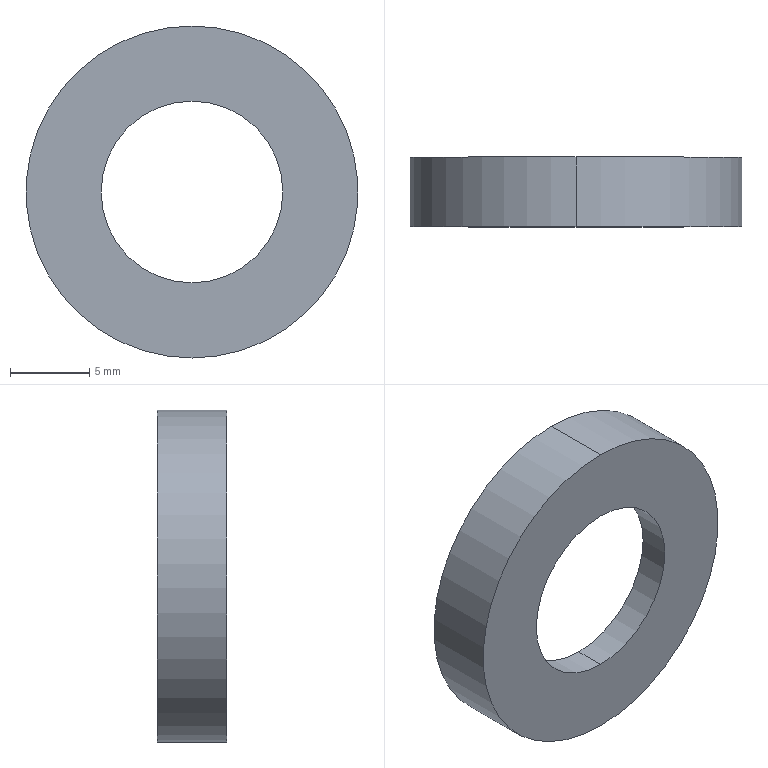Component | SolidWorks | SphericalWasherB21-1 | 1 solid | 8 faces | box 21 x 4.4 x 21 mm | volume 832 mm3 | cylinder 4 | cone 2 | plane 2 | commonest cylinder face diameters 21 x2 11.5 x2 | material Nickel
build123d program:
from build123d import *


with BuildPart() as part:
    # Sketch1 → Base-Revolve (revolve)
    with BuildSketch(Plane.XY, mode=Mode.PRIVATE) as base_revolve_sk:
        Polygon((5.75, 0), (10.5, 0), (10.5, 4.4), (10, 4.4), (5.75, 1.946), align=None)
    revolve(base_revolve_sk.sketch.rotate(Axis((0, 10.019, 0), (0, -1, 0)), 90), axis=Axis((0, 10.019, 0), (0, -1, 0)))


solid = part.part

# Placed as in the assembly
solid = solid.moved(Location((96, 228.606, 0), (0, 0, 0)))
STEP:
#1=COLOUR_RGB('',0.7922,0.8196,0.9333);
#2=FILL_AREA_STYLE_COLOUR('',#1);
#3=FILL_AREA_STYLE('',(#2));
#4=SURFACE_STYLE_FILL_AREA(#3);
#5=SURFACE_SIDE_STYLE('',(#4));
#6=SURFACE_STYLE_USAGE(.BOTH.,#5);
#7=PRESENTATION_STYLE_ASSIGNMENT((#6));
#8=CARTESIAN_POINT('',(3.78,9.077,-0.2264));
#9=VERTEX_POINT('',#8);
#10=CARTESIAN_POINT('',(3.78,9.077,0.2264));
#11=VERTEX_POINT('',#10);
#12=CARTESIAN_POINT('',(3.78,9.077,0.));
#13=DIRECTION('',(0.,1.,0.));
#14=DIRECTION('',(0.,0.,1.));
#15=AXIS2_PLACEMENT_3D('',#12,#13,#14);
#16=CIRCLE('',#15,0.2264);
#17=EDGE_CURVE('',#9,#11,#16,.T.);
#18=ORIENTED_EDGE('',*,*,#17,.F.);
#19=CARTESIAN_POINT('',(3.78,9.173,-0.3937));
#20=VERTEX_POINT('',#19);
#21=CARTESIAN_POINT('',(3.78,9.173,-0.3937));
#22=DIRECTION('',(0.,0.5,-0.866));
#23=VECTOR('',#22,39.37);
#24=LINE('',#21,#23);
#25=EDGE_CURVE('',#9,#20,#24,.T.);
#26=ORIENTED_EDGE('',*,*,#25,.T.);
#27=CARTESIAN_POINT('',(3.78,9.173,0.3937));
#28=VERTEX_POINT('',#27);
#29=CARTESIAN_POINT('',(3.78,9.173,0.));
#30=DIRECTION('',(0.,1.,0.));
#31=DIRECTION('',(0.,0.,1.));
#32=AXIS2_PLACEMENT_3D('',#29,#30,#31);
#33=CIRCLE('',#32,0.3937);
#34=EDGE_CURVE('',#20,#28,#33,.T.);
#35=ORIENTED_EDGE('',*,*,#34,.T.);
#36=CARTESIAN_POINT('',(3.78,9.173,0.3937));
#37=DIRECTION('',(0.,0.5,0.866));
#38=VECTOR('',#37,39.37);
#39=LINE('',#36,#38);
#40=EDGE_CURVE('',#11,#28,#39,.T.);
#41=ORIENTED_EDGE('',*,*,#40,.F.);
#42=EDGE_LOOP('',(#18,#26,#35,#41));
#43=FACE_OUTER_BOUND('',#42,.T.);
#44=CARTESIAN_POINT('',(3.78,9.173,0.));
#45=DIRECTION('',(0.,1.,0.));
#46=DIRECTION('',(0.,0.,1.));
#47=AXIS2_PLACEMENT_3D('',#44,#45,#46);
#48=CONICAL_SURFACE('',#47,0.3937,1.047);
#49=ADVANCED_FACE('',(#43),#48,.F.);
#50=CARTESIAN_POINT('',(3.78,9.,0.4134));
#51=VERTEX_POINT('',#50);
#52=CARTESIAN_POINT('',(3.78,9.,-0.4134));
#53=VERTEX_POINT('',#52);
#54=CARTESIAN_POINT('',(3.78,9.,0.));
#55=DIRECTION('',(0.,1.,0.));
#56=DIRECTION('',(0.,0.,1.));
#57=AXIS2_PLACEMENT_3D('',#54,#55,#56);
#58=CIRCLE('',#57,0.4134);
#59=EDGE_CURVE('',#51,#53,#58,.T.);
#60=ORIENTED_EDGE('',*,*,#59,.T.);
#61=CARTESIAN_POINT('',(3.78,9.173,-0.4134));
#62=VERTEX_POINT('',#61);
#63=CARTESIAN_POINT('',(3.78,9.395,-0.4134));
#64=DIRECTION('',(0.,1.,0.));
#65=VECTOR('',#64,39.37);
#66=LINE('',#63,#65);
#67=EDGE_CURVE('',#53,#62,#66,.T.);
#68=ORIENTED_EDGE('',*,*,#67,.T.);
#69=CARTESIAN_POINT('',(3.78,9.173,0.4134));
#70=VERTEX_POINT('',#69);
#71=CARTESIAN_POINT('',(3.78,9.173,0.));
#72=DIRECTION('',(0.,1.,0.));
#73=DIRECTION('',(0.,0.,1.));
#74=AXIS2_PLACEMENT_3D('',#71,#72,#73);
#75=CIRCLE('',#74,0.4134);
#76=EDGE_CURVE('',#70,#62,#75,.T.);
#77=ORIENTED_EDGE('',*,*,#76,.F.);
#78=CARTESIAN_POINT('',(3.78,9.395,0.4134));
#79=DIRECTION('',(0.,1.,0.));
#80=VECTOR('',#79,39.37);
#81=LINE('',#78,#80);
#82=EDGE_CURVE('',#51,#70,#81,.T.);
#83=ORIENTED_EDGE('',*,*,#82,.F.);
#84=EDGE_LOOP('',(#60,#68,#77,#83));
#85=FACE_OUTER_BOUND('',#84,.T.);
#86=CARTESIAN_POINT('',(3.78,9.395,0.));
#87=DIRECTION('',(0.,1.,0.));
#88=DIRECTION('',(0.,0.,1.));
#89=AXIS2_PLACEMENT_3D('',#86,#87,#88);
#90=CYLINDRICAL_SURFACE('',#89,0.4134);
#91=ADVANCED_FACE('',(#85),#90,.T.);
#92=CARTESIAN_POINT('',(3.78,9.,-0.2264));
#93=VERTEX_POINT('',#92);
#94=CARTESIAN_POINT('',(3.78,9.,0.2264));
#95=VERTEX_POINT('',#94);
#96=CARTESIAN_POINT('',(3.78,9.,0.));
#97=DIRECTION('',(0.,1.,0.));
#98=DIRECTION('',(0.,0.,1.));
#99=AXIS2_PLACEMENT_3D('',#96,#97,#98);
#100=CIRCLE('',#99,0.2264);
#101=EDGE_CURVE('',#93,#95,#100,.T.);
#102=ORIENTED_EDGE('',*,*,#101,.F.);
#103=CARTESIAN_POINT('',(3.78,9.395,-0.2264));
#104=DIRECTION('',(0.,1.,0.));
#105=VECTOR('',#104,39.37);
#106=LINE('',#103,#105);
#107=EDGE_CURVE('',#93,#9,#106,.T.);
#108=ORIENTED_EDGE('',*,*,#107,.T.);
#109=ORIENTED_EDGE('',*,*,#17,.T.);
#110=CARTESIAN_POINT('',(3.78,9.395,0.2264));
#111=DIRECTION('',(0.,1.,0.));
#112=VECTOR('',#111,39.37);
#113=LINE('',#110,#112);
#114=EDGE_CURVE('',#95,#11,#113,.T.);
#115=ORIENTED_EDGE('',*,*,#114,.F.);
#116=EDGE_LOOP('',(#102,#108,#109,#115));
#117=FACE_OUTER_BOUND('',#116,.T.);
#118=CARTESIAN_POINT('',(3.78,9.395,0.));
#119=DIRECTION('',(0.,1.,0.));
#120=DIRECTION('',(0.,0.,1.));
#121=AXIS2_PLACEMENT_3D('',#118,#119,#120);
#122=CYLINDRICAL_SURFACE('',#121,0.2264);
#123=ADVANCED_FACE('',(#117),#122,.F.);
#124=ORIENTED_EDGE('',*,*,#107,.F.);
#125=CARTESIAN_POINT('',(3.78,9.,0.));
#126=DIRECTION('',(0.,1.,0.));
#127=DIRECTION('',(0.,0.,1.));
#128=AXIS2_PLACEMENT_3D('',#125,#126,#127);
#129=CIRCLE('',#128,0.2264);
#130=EDGE_CURVE('',#95,#93,#129,.T.);
#131=ORIENTED_EDGE('',*,*,#130,.F.);
#132=ORIENTED_EDGE('',*,*,#114,.T.);
#133=CARTESIAN_POINT('',(3.78,9.077,0.));
#134=DIRECTION('',(0.,1.,0.));
#135=DIRECTION('',(0.,0.,1.));
#136=AXIS2_PLACEMENT_3D('',#133,#134,#135);
#137=CIRCLE('',#136,0.2264);
#138=EDGE_CURVE('',#11,#9,#137,.T.);
#139=ORIENTED_EDGE('',*,*,#138,.T.);
#140=EDGE_LOOP('',(#124,#131,#132,#139));
#141=FACE_OUTER_BOUND('',#140,.T.);
#142=CARTESIAN_POINT('',(3.78,9.395,0.));
#143=DIRECTION('',(0.,1.,0.));
#144=DIRECTION('',(0.,0.,1.));
#145=AXIS2_PLACEMENT_3D('',#142,#143,#144);
#146=CYLINDRICAL_SURFACE('',#145,0.2264);
#147=ADVANCED_FACE('',(#141),#146,.F.);
#148=ORIENTED_EDGE('',*,*,#59,.F.);
#149=CARTESIAN_POINT('',(3.78,9.,0.));
#150=DIRECTION('',(0.,1.,0.));
#151=DIRECTION('',(0.,0.,1.));
#152=AXIS2_PLACEMENT_3D('',#149,#150,#151);
#153=CIRCLE('',#152,0.4134);
#154=EDGE_CURVE('',#53,#51,#153,.T.);
#155=ORIENTED_EDGE('',*,*,#154,.F.);
#156=EDGE_LOOP('',(#148,#155));
#157=FACE_OUTER_BOUND('',#156,.T.);
#158=ORIENTED_EDGE('',*,*,#130,.T.);
#159=ORIENTED_EDGE('',*,*,#101,.T.);
#160=EDGE_LOOP('',(#158,#159));
#161=FACE_BOUND('',#160,.T.);
#162=CARTESIAN_POINT('',(4.006,9.,0.));
#163=DIRECTION('',(0.,1.,0.));
#164=DIRECTION('',(0.,0.,1.));
#165=AXIS2_PLACEMENT_3D('',#162,#163,#164);
#166=PLANE('',#165);
#167=ADVANCED_FACE('',(#157,#161),#166,.F.);
#168=ORIENTED_EDGE('',*,*,#67,.F.);
#169=ORIENTED_EDGE('',*,*,#154,.T.);
#170=ORIENTED_EDGE('',*,*,#82,.T.);
#171=CARTESIAN_POINT('',(3.78,9.173,0.));
#172=DIRECTION('',(0.,1.,0.));
#173=DIRECTION('',(0.,0.,1.));
#174=AXIS2_PLACEMENT_3D('',#171,#172,#173);
#175=CIRCLE('',#174,0.4134);
#176=EDGE_CURVE('',#62,#70,#175,.T.);
#177=ORIENTED_EDGE('',*,*,#176,.F.);
#178=EDGE_LOOP('',(#168,#169,#170,#177));
#179=FACE_OUTER_BOUND('',#178,.T.);
#180=CARTESIAN_POINT('',(3.78,9.395,0.));
#181=DIRECTION('',(0.,1.,0.));
#182=DIRECTION('',(0.,0.,1.));
#183=AXIS2_PLACEMENT_3D('',#180,#181,#182);
#184=CYLINDRICAL_SURFACE('',#183,0.4134);
#185=ADVANCED_FACE('',(#179),#184,.T.);
#186=CARTESIAN_POINT('',(3.78,9.173,0.));
#187=DIRECTION('',(0.,1.,0.));
#188=DIRECTION('',(0.,0.,1.));
#189=AXIS2_PLACEMENT_3D('',#186,#187,#188);
#190=CIRCLE('',#189,0.3937);
#191=EDGE_CURVE('',#28,#20,#190,.T.);
#192=ORIENTED_EDGE('',*,*,#191,.F.);
#193=ORIENTED_EDGE('',*,*,#34,.F.);
#194=EDGE_LOOP('',(#192,#193));
#195=FACE_BOUND('',#194,.T.);
#196=ORIENTED_EDGE('',*,*,#76,.T.);
#197=ORIENTED_EDGE('',*,*,#176,.T.);
#198=EDGE_LOOP('',(#196,#197));
#199=FACE_OUTER_BOUND('',#198,.T.);
#200=CARTESIAN_POINT('',(4.193,9.173,0.));
#201=DIRECTION('',(0.,-1.,0.));
#202=DIRECTION('',(0.,0.,-1.));
#203=AXIS2_PLACEMENT_3D('',#200,#201,#202);
#204=PLANE('',#203);
#205=ADVANCED_FACE('',(#195,#199),#204,.F.);
#206=ORIENTED_EDGE('',*,*,#25,.F.);
#207=ORIENTED_EDGE('',*,*,#138,.F.);
#208=ORIENTED_EDGE('',*,*,#40,.T.);
#209=ORIENTED_EDGE('',*,*,#191,.T.);
#210=EDGE_LOOP('',(#206,#207,#208,#209));
#211=FACE_OUTER_BOUND('',#210,.T.);
#212=CARTESIAN_POINT('',(3.78,9.173,0.));
#213=DIRECTION('',(0.,1.,0.));
#214=DIRECTION('',(0.,0.,1.));
#215=AXIS2_PLACEMENT_3D('',#212,#213,#214);
#216=CONICAL_SURFACE('',#215,0.3937,1.047);
#217=ADVANCED_FACE('',(#211),#216,.F.);
#218=CLOSED_SHELL('',(#49,#91,#123,#147,#167,#185,#205,#217));
#219=MANIFOLD_SOLID_BREP('',#218);
#220=STYLED_ITEM('',(#7),#219);
#221=PRESENTATION_LAYER_ASSIGNMENT('','',(#220));
#222=(LENGTH_UNIT()NAMED_UNIT(*)SI_UNIT($,.METRE.));
#223=LENGTH_MEASURE_WITH_UNIT(LENGTH_MEASURE(0.0254),#222);
#224=DIMENSIONAL_EXPONENTS(1.,0.,0.,0.,0.,0.,0.);
#225=(CONVERSION_BASED_UNIT('',#223)LENGTH_UNIT()NAMED_UNIT(#224));
#226=UNCERTAINTY_MEASURE_WITH_UNIT(LENGTH_MEASURE(0.00001),#225,'','');
#227=(NAMED_UNIT(*)PLANE_ANGLE_UNIT()SI_UNIT($,.RADIAN.));
#228=(NAMED_UNIT(*)SI_UNIT($,.STERADIAN.)SOLID_ANGLE_UNIT());
#229=(GEOMETRIC_REPRESENTATION_CONTEXT(3)GLOBAL_UNCERTAINTY_ASSIGNED_CONTEXT((#226))GLOBAL_UNIT_ASSIGNED_CONTEXT((#225,#227,#228))REPRESENTATION_CONTEXT('',''));
#230=MECHANICAL_DESIGN_GEOMETRIC_PRESENTATION_REPRESENTATION('',(#220),#229);
#231=CARTESIAN_POINT('',(0.,0.,0.));
#232=DIRECTION('',(0.,0.,1.));
#233=DIRECTION('',(1.,0.,0.));
#234=AXIS2_PLACEMENT_3D('',#231,#232,#233);
#235=(LENGTH_UNIT()NAMED_UNIT(*)SI_UNIT($,.METRE.));
#236=LENGTH_MEASURE_WITH_UNIT(LENGTH_MEASURE(0.0254),#235);
#237=DIMENSIONAL_EXPONENTS(1.,0.,0.,0.,0.,0.,0.);
#238=(CONVERSION_BASED_UNIT('',#236)LENGTH_UNIT()NAMED_UNIT(#237));
#239=UNCERTAINTY_MEASURE_WITH_UNIT(LENGTH_MEASURE(0.00001),#238,'','');
#240=(NAMED_UNIT(*)PLANE_ANGLE_UNIT()SI_UNIT($,.RADIAN.));
#241=(NAMED_UNIT(*)SI_UNIT($,.STERADIAN.)SOLID_ANGLE_UNIT());
#242=(GEOMETRIC_REPRESENTATION_CONTEXT(3)GLOBAL_UNCERTAINTY_ASSIGNED_CONTEXT((#239))GLOBAL_UNIT_ASSIGNED_CONTEXT((#238,#240,#241))REPRESENTATION_CONTEXT('',''));
#243=ADVANCED_BREP_SHAPE_REPRESENTATION('',(#219,#234),#242);